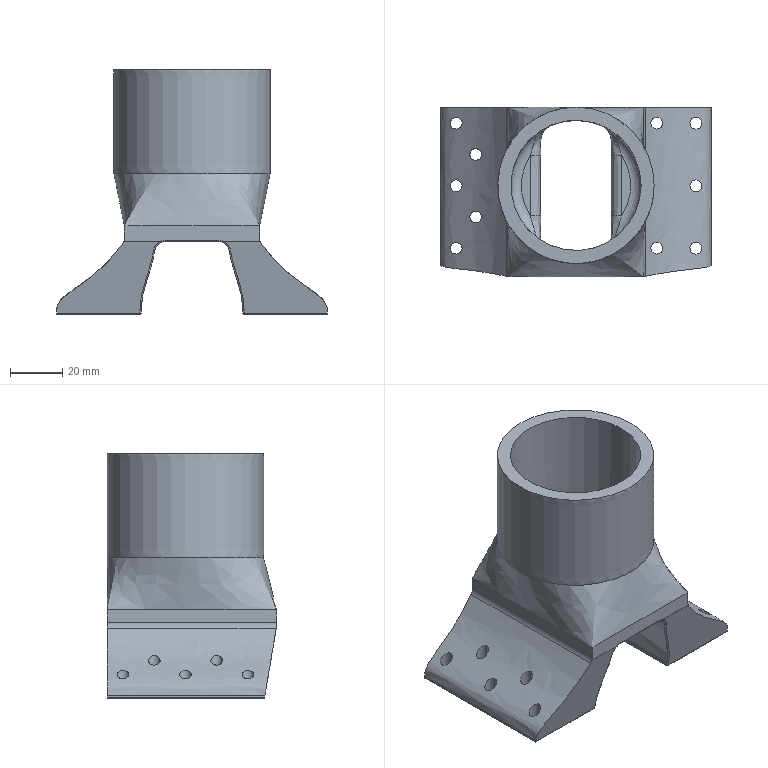Component | NX | TILT_ROTORROD_CONN_MNT | 1 solid | 100 faces | volume 143180 mm3 | plane 33 | cylinder 32 | spline 19 | torus 6 | other 5 | sphere 5 | commonest cylinder face diameters 1 x15 4.5 x10 8 x6 50 x1